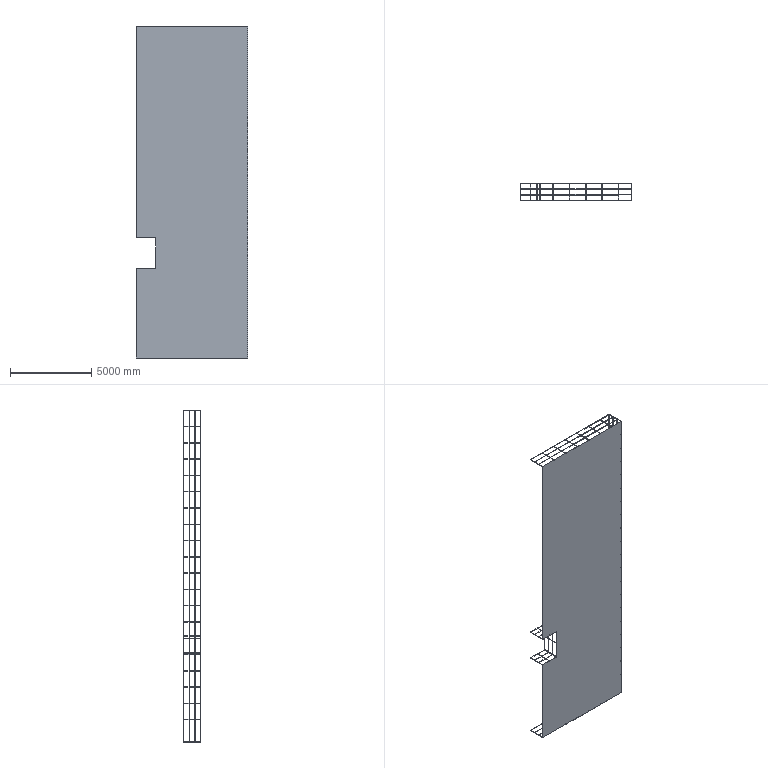Component | NX | Root-owned geometry | 61 solids | 389 faces | volume 891446833 mm3 | plane 197 | cylinder 192 | commonest cylinder face diameters 20 x150 32 x42